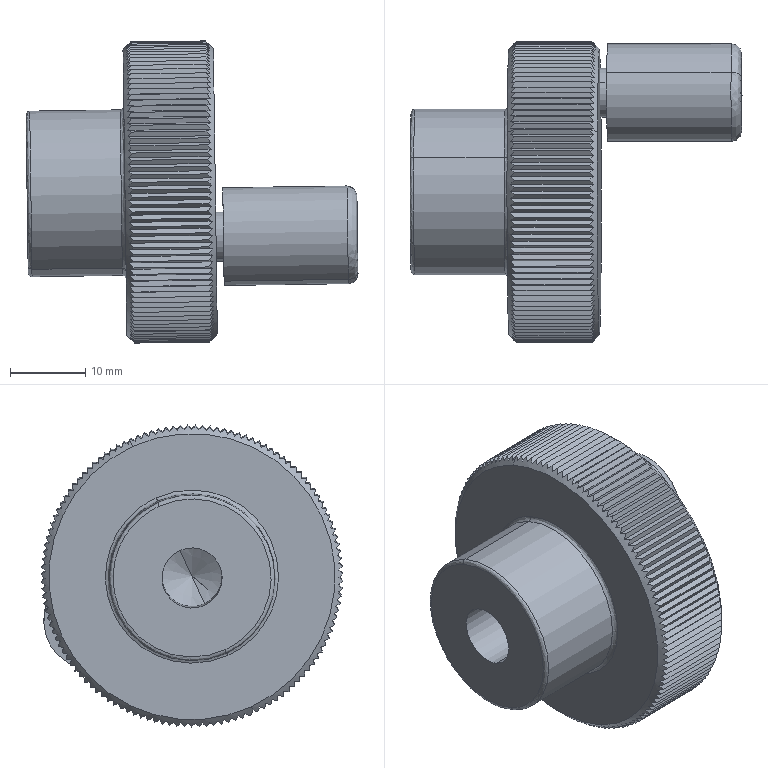Component | SolidWorks | DA-0220-HBK40-4 | 1 solid | 299 faces | volume 21115 mm3 | plane 268 | cylinder 14 | spline 11 | cone 6 | commonest cylinder face diameters 8.267 x3 6.5 x2 13 x2 8.667 x2 22 x2 8 x2 40 x1